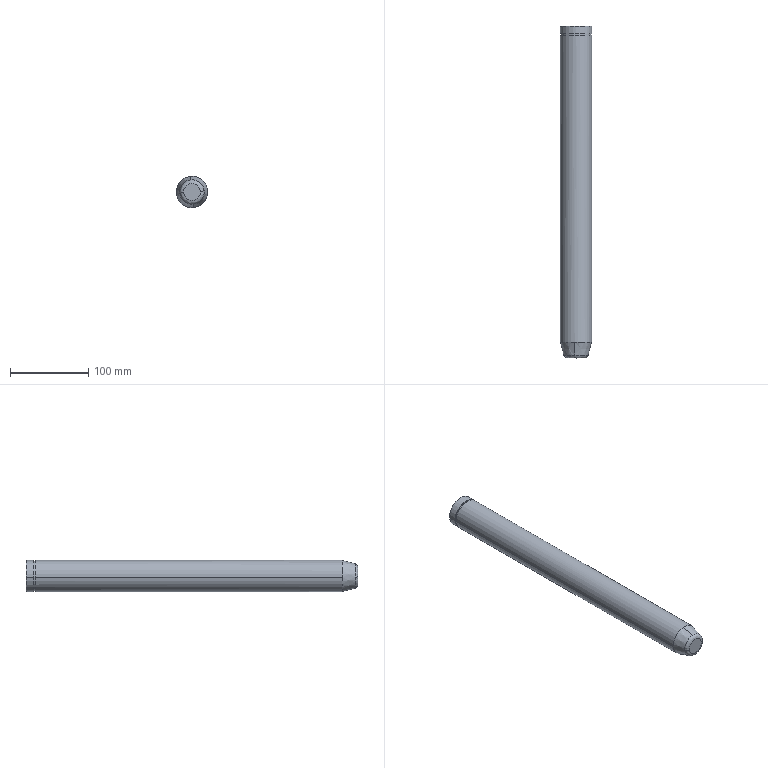Component | SolidWorks | YC1-250-05-02EjectorRod-1 | 1 solid | 14 faces | box 40 x 425 x 40 mm | volume 527461 mm3 | cylinder 6 | plane 4 | spline 2 | cone 2 | commonest cylinder face diameters 40 x4 38 x2 | material Plain Carbon Steel
STEP:
#1=CARTESIAN_POINT('',(-24.636,78.351,-0.05895));
#2=VERTEX_POINT('',#1);
#3=CARTESIAN_POINT('',(-23.789,78.351,0.01958));
#4=VERTEX_POINT('',#3);
#5=CARTESIAN_POINT('',(-24.636,78.351,-0.05895));
#6=CARTESIAN_POINT('',(-24.715,78.351,0.7882));
#7=CARTESIAN_POINT('',(-23.868,78.351,0.8667));
#8=CARTESIAN_POINT('',(-23.789,78.351,0.01958));
#9=(BOUNDED_CURVE()B_SPLINE_CURVE(3,(#5,#6,#7,#8),.UNSPECIFIED.,.F.,.F.)B_SPLINE_CURVE_WITH_KNOTS((4,4),(0.,1.),.UNSPECIFIED.)CURVE()GEOMETRIC_REPRESENTATION_ITEM()RATIONAL_B_SPLINE_CURVE((1.,0.3333,0.3333,1.))REPRESENTATION_ITEM(''));
#10=EDGE_CURVE('',#2,#4,#9,.T.);
#11=ORIENTED_EDGE('',*,*,#10,.T.);
#12=CARTESIAN_POINT('',(-23.6,78.497,0.03714));
#13=VERTEX_POINT('',#12);
#14=CARTESIAN_POINT('',(-23.789,78.547,0.01958));
#15=DIRECTION('',(-0.09232,0.,0.9957));
#16=DIRECTION('',(0.9957,0.,0.09232));
#17=AXIS2_PLACEMENT_3D('',#14,#15,#16);
#18=CIRCLE('',#17,0.1969);
#19=EDGE_CURVE('',#4,#13,#18,.T.);
#20=ORIENTED_EDGE('',*,*,#19,.T.);
#21=CARTESIAN_POINT('',(-24.269,78.497,0.5932));
#22=VERTEX_POINT('',#21);
#23=CARTESIAN_POINT('',(-24.213,78.497,-0.01969));
#24=DIRECTION('',(0.,1.,0.));
#25=DIRECTION('',(0.9957,0.,0.09232));
#26=AXIS2_PLACEMENT_3D('',#23,#24,#25);
#27=CIRCLE('',#26,0.6155);
#28=EDGE_CURVE('',#22,#13,#27,.T.);
#29=ORIENTED_EDGE('',*,*,#28,.F.);
#30=CARTESIAN_POINT('',(-24.825,78.497,-0.07651));
#31=VERTEX_POINT('',#30);
#32=CARTESIAN_POINT('',(-24.213,78.497,-0.01969));
#33=DIRECTION('',(0.,1.,0.));
#34=DIRECTION('',(0.9957,0.,0.09232));
#35=AXIS2_PLACEMENT_3D('',#32,#33,#34);
#36=CIRCLE('',#35,0.6155);
#37=EDGE_CURVE('',#31,#22,#36,.T.);
#38=ORIENTED_EDGE('',*,*,#37,.F.);
#39=CARTESIAN_POINT('',(-24.636,78.547,-0.05895));
#40=DIRECTION('',(0.09232,0.,-0.9957));
#41=DIRECTION('',(-0.9957,0.,-0.09232));
#42=AXIS2_PLACEMENT_3D('',#39,#40,#41);
#43=CIRCLE('',#42,0.1969);
#44=EDGE_CURVE('',#2,#31,#43,.T.);
#45=ORIENTED_EDGE('',*,*,#44,.F.);
#46=EDGE_LOOP('',(#11,#20,#29,#38,#45));
#47=FACE_OUTER_BOUND('',#46,.T.);
#48=CARTESIAN_POINT('',(-23.789,78.351,0.01958));
#49=CARTESIAN_POINT('',(-23.868,78.351,0.8667));
#50=CARTESIAN_POINT('',(-24.715,78.351,0.7882));
#51=CARTESIAN_POINT('',(-24.636,78.351,-0.05895));
#52=CARTESIAN_POINT('',(-23.697,78.351,0.02814));
#53=CARTESIAN_POINT('',(-23.792,78.351,1.06));
#54=CARTESIAN_POINT('',(-24.824,78.351,0.9641));
#55=CARTESIAN_POINT('',(-24.728,78.351,-0.06751));
#56=CARTESIAN_POINT('',(-23.624,78.407,0.03492));
#57=CARTESIAN_POINT('',(-23.733,78.407,1.213));
#58=CARTESIAN_POINT('',(-24.911,78.407,1.104));
#59=CARTESIAN_POINT('',(-24.802,78.407,-0.07429));
#60=CARTESIAN_POINT('',(-23.6,78.497,0.03714));
#61=CARTESIAN_POINT('',(-23.713,78.497,1.263));
#62=CARTESIAN_POINT('',(-24.939,78.497,1.149));
#63=CARTESIAN_POINT('',(-24.825,78.497,-0.07651));
#64=(BOUNDED_SURFACE()B_SPLINE_SURFACE(3,3,((#48,#49,#50,#51),(#52,#53,#54,#55),(#56,#57,#58,#59),(#60,#61,#62,#63)),.UNSPECIFIED.,.F.,.F.,.F.)B_SPLINE_SURFACE_WITH_KNOTS((4,4),(4,4),(0.,1.),(0.,1.),.UNSPECIFIED.)GEOMETRIC_REPRESENTATION_ITEM()RATIONAL_B_SPLINE_SURFACE(((1.,0.3333,0.3333,1.),(0.8622,0.2874,0.2874,0.8622),(0.8622,0.2874,0.2874,0.8622),(1.,0.3333,0.3333,1.)))REPRESENTATION_ITEM('')SURFACE());
#65=ADVANCED_FACE('',(#47),#64,.T.);
#66=CARTESIAN_POINT('',(-24.997,94.614,-0.09237));
#67=VERTEX_POINT('',#66);
#68=CARTESIAN_POINT('',(-23.429,94.614,0.053));
#69=VERTEX_POINT('',#68);
#70=CARTESIAN_POINT('',(-24.213,94.614,-0.01969));
#71=DIRECTION('',(0.,-1.,0.));
#72=DIRECTION('',(-0.9957,0.,-0.09232));
#73=AXIS2_PLACEMENT_3D('',#70,#71,#72);
#74=CIRCLE('',#73,0.7874);
#75=EDGE_CURVE('',#67,#69,#74,.T.);
#76=ORIENTED_EDGE('',*,*,#75,.T.);
#77=CARTESIAN_POINT('',(-23.429,79.138,0.053));
#78=VERTEX_POINT('',#77);
#79=CARTESIAN_POINT('',(-23.429,78.351,0.053));
#80=DIRECTION('',(0.,-1.,0.));
#81=VECTOR('',#80,39.37);
#82=LINE('',#79,#81);
#83=EDGE_CURVE('',#69,#78,#82,.T.);
#84=ORIENTED_EDGE('',*,*,#83,.T.);
#85=CARTESIAN_POINT('',(-24.14,79.138,-0.8037));
#86=VERTEX_POINT('',#85);
#87=CARTESIAN_POINT('',(-24.213,79.138,-0.01969));
#88=DIRECTION('',(0.,1.,0.));
#89=DIRECTION('',(-0.9957,0.,-0.09232));
#90=AXIS2_PLACEMENT_3D('',#87,#88,#89);
#91=CIRCLE('',#90,0.7874);
#92=EDGE_CURVE('',#78,#86,#91,.T.);
#93=ORIENTED_EDGE('',*,*,#92,.T.);
#94=CARTESIAN_POINT('',(-24.997,79.138,-0.09237));
#95=VERTEX_POINT('',#94);
#96=CARTESIAN_POINT('',(-24.213,79.138,-0.01969));
#97=DIRECTION('',(0.,1.,0.));
#98=DIRECTION('',(-0.9957,0.,-0.09232));
#99=AXIS2_PLACEMENT_3D('',#96,#97,#98);
#100=CIRCLE('',#99,0.7874);
#101=EDGE_CURVE('',#86,#95,#100,.T.);
#102=ORIENTED_EDGE('',*,*,#101,.T.);
#103=CARTESIAN_POINT('',(-24.997,78.351,-0.09237));
#104=DIRECTION('',(0.,-1.,0.));
#105=VECTOR('',#104,39.37);
#106=LINE('',#103,#105);
#107=EDGE_CURVE('',#67,#95,#106,.T.);
#108=ORIENTED_EDGE('',*,*,#107,.F.);
#109=EDGE_LOOP('',(#76,#84,#93,#102,#108));
#110=FACE_OUTER_BOUND('',#109,.T.);
#111=CARTESIAN_POINT('',(-24.213,78.351,-0.01969));
#112=DIRECTION('',(0.,-1.,0.));
#113=DIRECTION('',(-0.9957,0.,-0.09232));
#114=AXIS2_PLACEMENT_3D('',#111,#112,#113);
#115=CYLINDRICAL_SURFACE('',#114,0.7874);
#116=ADVANCED_FACE('',(#110),#115,.T.);
#117=ORIENTED_EDGE('',*,*,#28,.T.);
#118=CARTESIAN_POINT('',(-24.156,78.497,-0.6326));
#119=VERTEX_POINT('',#118);
#120=CARTESIAN_POINT('',(-24.213,78.497,-0.01969));
#121=DIRECTION('',(0.,1.,0.));
#122=DIRECTION('',(0.9957,0.,0.09232));
#123=AXIS2_PLACEMENT_3D('',#120,#121,#122);
#124=CIRCLE('',#123,0.6155);
#125=EDGE_CURVE('',#13,#119,#124,.T.);
#126=ORIENTED_EDGE('',*,*,#125,.T.);
#127=CARTESIAN_POINT('',(-24.14,79.138,-0.8037));
#128=DIRECTION('',(0.02389,0.9659,-0.2577));
#129=VECTOR('',#128,39.37);
#130=LINE('',#127,#129);
#131=EDGE_CURVE('',#119,#86,#130,.T.);
#132=ORIENTED_EDGE('',*,*,#131,.T.);
#133=ORIENTED_EDGE('',*,*,#92,.F.);
#134=CARTESIAN_POINT('',(-24.285,79.138,0.7644));
#135=VERTEX_POINT('',#134);
#136=CARTESIAN_POINT('',(-24.213,79.138,-0.01969));
#137=DIRECTION('',(0.,1.,0.));
#138=DIRECTION('',(-0.9957,0.,-0.09232));
#139=AXIS2_PLACEMENT_3D('',#136,#137,#138);
#140=CIRCLE('',#139,0.7874);
#141=EDGE_CURVE('',#135,#78,#140,.T.);
#142=ORIENTED_EDGE('',*,*,#141,.F.);
#143=CARTESIAN_POINT('',(-24.285,79.138,0.7644));
#144=DIRECTION('',(-0.02389,0.9659,0.2577));
#145=VECTOR('',#144,39.37);
#146=LINE('',#143,#145);
#147=EDGE_CURVE('',#22,#135,#146,.T.);
#148=ORIENTED_EDGE('',*,*,#147,.F.);
#149=EDGE_LOOP('',(#117,#126,#132,#133,#142,#148));
#150=FACE_OUTER_BOUND('',#149,.T.);
#151=CARTESIAN_POINT('',(-24.213,79.138,-0.01969));
#152=DIRECTION('',(0.,1.,-0.));
#153=DIRECTION('',(-0.09232,0.,0.9957));
#154=AXIS2_PLACEMENT_3D('',#151,#152,#153);
#155=CONICAL_SURFACE('',#154,0.7874,0.2618);
#156=ADVANCED_FACE('',(#150),#155,.T.);
#157=CARTESIAN_POINT('',(-24.957,94.689,-0.08874));
#158=VERTEX_POINT('',#157);
#159=CARTESIAN_POINT('',(-23.468,94.689,0.04937));
#160=VERTEX_POINT('',#159);
#161=CARTESIAN_POINT('',(-24.213,94.689,-0.01969));
#162=DIRECTION('',(0.,-1.,0.));
#163=DIRECTION('',(-0.9957,0.,-0.09232));
#164=AXIS2_PLACEMENT_3D('',#161,#162,#163);
#165=CIRCLE('',#164,0.748);
#166=EDGE_CURVE('',#158,#160,#165,.T.);
#167=ORIENTED_EDGE('',*,*,#166,.T.);
#168=CARTESIAN_POINT('',(-23.468,94.614,0.04937));
#169=VERTEX_POINT('',#168);
#170=CARTESIAN_POINT('',(-23.468,78.351,0.04937));
#171=DIRECTION('',(0.,-1.,0.));
#172=VECTOR('',#171,39.37);
#173=LINE('',#170,#172);
#174=EDGE_CURVE('',#160,#169,#173,.T.);
#175=ORIENTED_EDGE('',*,*,#174,.T.);
#176=CARTESIAN_POINT('',(-24.957,94.614,-0.08874));
#177=VERTEX_POINT('',#176);
#178=CARTESIAN_POINT('',(-24.213,94.614,-0.01969));
#179=DIRECTION('',(0.,1.,0.));
#180=DIRECTION('',(-0.9957,0.,-0.09232));
#181=AXIS2_PLACEMENT_3D('',#178,#179,#180);
#182=CIRCLE('',#181,0.748);
#183=EDGE_CURVE('',#169,#177,#182,.T.);
#184=ORIENTED_EDGE('',*,*,#183,.T.);
#185=CARTESIAN_POINT('',(-24.957,78.351,-0.08874));
#186=DIRECTION('',(0.,-1.,0.));
#187=VECTOR('',#186,39.37);
#188=LINE('',#185,#187);
#189=EDGE_CURVE('',#158,#177,#188,.T.);
#190=ORIENTED_EDGE('',*,*,#189,.F.);
#191=EDGE_LOOP('',(#167,#175,#184,#190));
#192=FACE_OUTER_BOUND('',#191,.T.);
#193=CARTESIAN_POINT('',(-24.213,78.351,-0.01969));
#194=DIRECTION('',(0.,-1.,0.));
#195=DIRECTION('',(-0.9957,0.,-0.09232));
#196=AXIS2_PLACEMENT_3D('',#193,#194,#195);
#197=CYLINDRICAL_SURFACE('',#196,0.748);
#198=ADVANCED_FACE('',(#192),#197,.T.);
#199=CARTESIAN_POINT('',(-24.997,95.083,-0.09237));
#200=VERTEX_POINT('',#199);
#201=CARTESIAN_POINT('',(-23.429,95.083,0.053));
#202=VERTEX_POINT('',#201);
#203=CARTESIAN_POINT('',(-24.213,95.083,-0.01969));
#204=DIRECTION('',(0.,-1.,0.));
#205=DIRECTION('',(-0.9957,0.,-0.09232));
#206=AXIS2_PLACEMENT_3D('',#203,#204,#205);
#207=CIRCLE('',#206,0.7874);
#208=EDGE_CURVE('',#200,#202,#207,.T.);
#209=ORIENTED_EDGE('',*,*,#208,.T.);
#210=CARTESIAN_POINT('',(-23.429,94.689,0.053));
#211=VERTEX_POINT('',#210);
#212=CARTESIAN_POINT('',(-23.429,78.351,0.053));
#213=DIRECTION('',(0.,-1.,0.));
#214=VECTOR('',#213,39.37);
#215=LINE('',#212,#214);
#216=EDGE_CURVE('',#202,#211,#215,.T.);
#217=ORIENTED_EDGE('',*,*,#216,.T.);
#218=CARTESIAN_POINT('',(-24.997,94.689,-0.09237));
#219=VERTEX_POINT('',#218);
#220=CARTESIAN_POINT('',(-24.213,94.689,-0.01969));
#221=DIRECTION('',(0.,1.,0.));
#222=DIRECTION('',(-0.9957,0.,-0.09232));
#223=AXIS2_PLACEMENT_3D('',#220,#221,#222);
#224=CIRCLE('',#223,0.7874);
#225=EDGE_CURVE('',#211,#219,#224,.T.);
#226=ORIENTED_EDGE('',*,*,#225,.T.);
#227=CARTESIAN_POINT('',(-24.997,78.351,-0.09237));
#228=DIRECTION('',(0.,-1.,0.));
#229=VECTOR('',#228,39.37);
#230=LINE('',#227,#229);
#231=EDGE_CURVE('',#200,#219,#230,.T.);
#232=ORIENTED_EDGE('',*,*,#231,.F.);
#233=EDGE_LOOP('',(#209,#217,#226,#232));
#234=FACE_OUTER_BOUND('',#233,.T.);
#235=CARTESIAN_POINT('',(-24.213,78.351,-0.01969));
#236=DIRECTION('',(0.,-1.,0.));
#237=DIRECTION('',(-0.9957,0.,-0.09232));
#238=AXIS2_PLACEMENT_3D('',#235,#236,#237);
#239=CYLINDRICAL_SURFACE('',#238,0.7874);
#240=ADVANCED_FACE('',(#234),#239,.T.);
#241=ORIENTED_EDGE('',*,*,#83,.F.);
#242=CARTESIAN_POINT('',(-24.213,94.614,-0.01969));
#243=DIRECTION('',(0.,-1.,0.));
#244=DIRECTION('',(-0.9957,0.,-0.09232));
#245=AXIS2_PLACEMENT_3D('',#242,#243,#244);
#246=CIRCLE('',#245,0.7874);
#247=EDGE_CURVE('',#69,#67,#246,.T.);
#248=ORIENTED_EDGE('',*,*,#247,.T.);
#249=ORIENTED_EDGE('',*,*,#107,.T.);
#250=CARTESIAN_POINT('',(-24.213,79.138,-0.01969));
#251=DIRECTION('',(0.,1.,0.));
#252=DIRECTION('',(-0.9957,0.,-0.09232));
#253=AXIS2_PLACEMENT_3D('',#250,#251,#252);
#254=CIRCLE('',#253,0.7874);
#255=EDGE_CURVE('',#95,#135,#254,.T.);
#256=ORIENTED_EDGE('',*,*,#255,.T.);
#257=ORIENTED_EDGE('',*,*,#141,.T.);
#258=EDGE_LOOP('',(#241,#248,#249,#256,#257));
#259=FACE_OUTER_BOUND('',#258,.T.);
#260=CARTESIAN_POINT('',(-24.213,78.351,-0.01969));
#261=DIRECTION('',(0.,-1.,0.));
#262=DIRECTION('',(-0.9957,0.,-0.09232));
#263=AXIS2_PLACEMENT_3D('',#260,#261,#262);
#264=CYLINDRICAL_SURFACE('',#263,0.7874);
#265=ADVANCED_FACE('',(#259),#264,.T.);
#266=ORIENTED_EDGE('',*,*,#131,.F.);
#267=CARTESIAN_POINT('',(-24.213,78.497,-0.01969));
#268=DIRECTION('',(0.,1.,0.));
#269=DIRECTION('',(0.9957,0.,0.09232));
#270=AXIS2_PLACEMENT_3D('',#267,#268,#269);
#271=CIRCLE('',#270,0.6155);
#272=EDGE_CURVE('',#119,#31,#271,.T.);
#273=ORIENTED_EDGE('',*,*,#272,.T.);
#274=ORIENTED_EDGE('',*,*,#37,.T.);
#275=ORIENTED_EDGE('',*,*,#147,.T.);
#276=ORIENTED_EDGE('',*,*,#255,.F.);
#277=ORIENTED_EDGE('',*,*,#101,.F.);
#278=EDGE_LOOP('',(#266,#273,#274,#275,#276,#277));
#279=FACE_OUTER_BOUND('',#278,.T.);
#280=CARTESIAN_POINT('',(-24.213,79.138,-0.01969));
#281=DIRECTION('',(0.,1.,-0.));
#282=DIRECTION('',(-0.09232,0.,0.9957));
#283=AXIS2_PLACEMENT_3D('',#280,#281,#282);
#284=CONICAL_SURFACE('',#283,0.7874,0.2618);
#285=ADVANCED_FACE('',(#279),#284,.T.);
#286=CARTESIAN_POINT('',(-24.213,94.614,-0.01969));
#287=DIRECTION('',(0.,1.,0.));
#288=DIRECTION('',(-0.9957,0.,-0.09232));
#289=AXIS2_PLACEMENT_3D('',#286,#287,#288);
#290=CIRCLE('',#289,0.748);
#291=EDGE_CURVE('',#177,#169,#290,.T.);
#292=ORIENTED_EDGE('',*,*,#291,.F.);
#293=ORIENTED_EDGE('',*,*,#183,.F.);
#294=EDGE_LOOP('',(#292,#293));
#295=FACE_BOUND('',#294,.T.);
#296=ORIENTED_EDGE('',*,*,#75,.F.);
#297=ORIENTED_EDGE('',*,*,#247,.F.);
#298=EDGE_LOOP('',(#296,#297));
#299=FACE_OUTER_BOUND('',#298,.T.);
#300=CARTESIAN_POINT('',(-24.144,94.614,-0.7645));
#301=DIRECTION('',(0.,-1.,0.));
#302=DIRECTION('',(-0.9957,0.,-0.09232));
#303=AXIS2_PLACEMENT_3D('',#300,#301,#302);
#304=PLANE('',#303);
#305=ADVANCED_FACE('',(#295,#299),#304,.F.);
#306=ORIENTED_EDGE('',*,*,#19,.F.);
#307=CARTESIAN_POINT('',(-23.789,78.351,0.01958));
#308=CARTESIAN_POINT('',(-23.711,78.351,-0.8275));
#309=CARTESIAN_POINT('',(-24.558,78.351,-0.9061));
#310=CARTESIAN_POINT('',(-24.636,78.351,-0.05895));
#311=(BOUNDED_CURVE()B_SPLINE_CURVE(3,(#307,#308,#309,#310),.UNSPECIFIED.,.F.,.T.)B_SPLINE_CURVE_WITH_KNOTS((4,4),(0.,1.),.UNSPECIFIED.)CURVE()GEOMETRIC_REPRESENTATION_ITEM()RATIONAL_B_SPLINE_CURVE((1.,0.3333,0.3333,1.))REPRESENTATION_ITEM(''));
#312=EDGE_CURVE('',#4,#2,#311,.T.);
#313=ORIENTED_EDGE('',*,*,#312,.T.);
#314=ORIENTED_EDGE('',*,*,#44,.T.);
#315=ORIENTED_EDGE('',*,*,#272,.F.);
#316=ORIENTED_EDGE('',*,*,#125,.F.);
#317=EDGE_LOOP('',(#306,#313,#314,#315,#316));
#318=FACE_OUTER_BOUND('',#317,.T.);
#319=CARTESIAN_POINT('',(-24.636,78.351,-0.05895));
#320=CARTESIAN_POINT('',(-24.558,78.351,-0.9061));
#321=CARTESIAN_POINT('',(-23.711,78.351,-0.8275));
#322=CARTESIAN_POINT('',(-23.789,78.351,0.01958));
#323=CARTESIAN_POINT('',(-24.728,78.351,-0.06751));
#324=CARTESIAN_POINT('',(-24.633,78.351,-1.099));
#325=CARTESIAN_POINT('',(-23.601,78.351,-1.003));
#326=CARTESIAN_POINT('',(-23.697,78.351,0.02814));
#327=CARTESIAN_POINT('',(-24.802,78.407,-0.07429));
#328=CARTESIAN_POINT('',(-24.692,78.407,-1.252));
#329=CARTESIAN_POINT('',(-23.514,78.407,-1.143));
#330=CARTESIAN_POINT('',(-23.624,78.407,0.03492));
#331=CARTESIAN_POINT('',(-24.825,78.497,-0.07651));
#332=CARTESIAN_POINT('',(-24.712,78.497,-1.302));
#333=CARTESIAN_POINT('',(-23.486,78.497,-1.189));
#334=CARTESIAN_POINT('',(-23.6,78.497,0.03714));
#335=(BOUNDED_SURFACE()B_SPLINE_SURFACE(3,3,((#319,#320,#321,#322),(#323,#324,#325,#326),(#327,#328,#329,#330),(#331,#332,#333,#334)),.UNSPECIFIED.,.F.,.F.,.F.)B_SPLINE_SURFACE_WITH_KNOTS((4,4),(4,4),(0.,1.),(0.,1.),.UNSPECIFIED.)GEOMETRIC_REPRESENTATION_ITEM()RATIONAL_B_SPLINE_SURFACE(((1.,0.3333,0.3333,1.),(0.8622,0.2874,0.2874,0.8622),(0.8622,0.2874,0.2874,0.8622),(1.,0.3333,0.3333,1.)))REPRESENTATION_ITEM('')SURFACE());
#336=ADVANCED_FACE('',(#318),#335,.T.);
#337=ORIENTED_EDGE('',*,*,#174,.F.);
#338=CARTESIAN_POINT('',(-24.213,94.689,-0.01969));
#339=DIRECTION('',(0.,-1.,0.));
#340=DIRECTION('',(-0.9957,0.,-0.09232));
#341=AXIS2_PLACEMENT_3D('',#338,#339,#340);
#342=CIRCLE('',#341,0.748);
#343=EDGE_CURVE('',#160,#158,#342,.T.);
#344=ORIENTED_EDGE('',*,*,#343,.T.);
#345=ORIENTED_EDGE('',*,*,#189,.T.);
#346=ORIENTED_EDGE('',*,*,#291,.T.);
#347=EDGE_LOOP('',(#337,#344,#345,#346));
#348=FACE_OUTER_BOUND('',#347,.T.);
#349=CARTESIAN_POINT('',(-24.213,78.351,-0.01969));
#350=DIRECTION('',(0.,-1.,0.));
#351=DIRECTION('',(-0.9957,0.,-0.09232));
#352=AXIS2_PLACEMENT_3D('',#349,#350,#351);
#353=CYLINDRICAL_SURFACE('',#352,0.748);
#354=ADVANCED_FACE('',(#348),#353,.T.);
#355=ORIENTED_EDGE('',*,*,#312,.F.);
#356=ORIENTED_EDGE('',*,*,#10,.F.);
#357=EDGE_LOOP('',(#355,#356));
#358=FACE_OUTER_BOUND('',#357,.T.);
#359=CARTESIAN_POINT('',(-24.213,78.351,-0.01969));
#360=DIRECTION('',(0.,-1.,0.));
#361=DIRECTION('',(-0.9957,0.,-0.09232));
#362=AXIS2_PLACEMENT_3D('',#359,#360,#361);
#363=PLANE('',#362);
#364=ADVANCED_FACE('',(#358),#363,.T.);
#365=CARTESIAN_POINT('',(-24.213,94.689,-0.01969));
#366=DIRECTION('',(0.,1.,0.));
#367=DIRECTION('',(-0.9957,0.,-0.09232));
#368=AXIS2_PLACEMENT_3D('',#365,#366,#367);
#369=CIRCLE('',#368,0.7874);
#370=EDGE_CURVE('',#219,#211,#369,.T.);
#371=ORIENTED_EDGE('',*,*,#370,.F.);
#372=ORIENTED_EDGE('',*,*,#225,.F.);
#373=EDGE_LOOP('',(#371,#372));
#374=FACE_OUTER_BOUND('',#373,.T.);
#375=ORIENTED_EDGE('',*,*,#166,.F.);
#376=ORIENTED_EDGE('',*,*,#343,.F.);
#377=EDGE_LOOP('',(#375,#376));
#378=FACE_BOUND('',#377,.T.);
#379=CARTESIAN_POINT('',(-24.144,94.689,-0.7645));
#380=DIRECTION('',(0.,1.,0.));
#381=DIRECTION('',(0.9957,0.,0.09232));
#382=AXIS2_PLACEMENT_3D('',#379,#380,#381);
#383=PLANE('',#382);
#384=ADVANCED_FACE('',(#374,#378),#383,.F.);
#385=ORIENTED_EDGE('',*,*,#216,.F.);
#386=CARTESIAN_POINT('',(-24.213,95.083,-0.01969));
#387=DIRECTION('',(0.,-1.,0.));
#388=DIRECTION('',(-0.9957,0.,-0.09232));
#389=AXIS2_PLACEMENT_3D('',#386,#387,#388);
#390=CIRCLE('',#389,0.7874);
#391=EDGE_CURVE('',#202,#200,#390,.T.);
#392=ORIENTED_EDGE('',*,*,#391,.T.);
#393=ORIENTED_EDGE('',*,*,#231,.T.);
#394=ORIENTED_EDGE('',*,*,#370,.T.);
#395=EDGE_LOOP('',(#385,#392,#393,#394));
#396=FACE_OUTER_BOUND('',#395,.T.);
#397=CARTESIAN_POINT('',(-24.213,78.351,-0.01969));
#398=DIRECTION('',(0.,-1.,0.));
#399=DIRECTION('',(-0.9957,0.,-0.09232));
#400=AXIS2_PLACEMENT_3D('',#397,#398,#399);
#401=CYLINDRICAL_SURFACE('',#400,0.7874);
#402=ADVANCED_FACE('',(#396),#401,.T.);
#403=ORIENTED_EDGE('',*,*,#208,.F.);
#404=ORIENTED_EDGE('',*,*,#391,.F.);
#405=EDGE_LOOP('',(#403,#404));
#406=FACE_OUTER_BOUND('',#405,.T.);
#407=CARTESIAN_POINT('',(-24.14,95.083,-0.8037));
#408=DIRECTION('',(0.,1.,0.));
#409=DIRECTION('',(0.9957,0.,0.09232));
#410=AXIS2_PLACEMENT_3D('',#407,#408,#409);
#411=PLANE('',#410);
#412=ADVANCED_FACE('',(#406),#411,.T.);
#413=CLOSED_SHELL('',(#65,#116,#156,#198,#240,#265,#285,#305,#336,#354,#364,#384,#402,#412));
#414=MANIFOLD_SOLID_BREP('',#413);
#415=CARTESIAN_POINT('',(0.,0.,0.));
#416=DIRECTION('',(0.,0.,1.));
#417=DIRECTION('',(1.,0.,0.));
#418=AXIS2_PLACEMENT_3D('',#415,#416,#417);
#419=(LENGTH_UNIT()NAMED_UNIT(*)SI_UNIT($,.METRE.));
#420=LENGTH_MEASURE_WITH_UNIT(LENGTH_MEASURE(0.0254),#419);
#421=DIMENSIONAL_EXPONENTS(1.,0.,0.,0.,0.,0.,0.);
#422=(CONVERSION_BASED_UNIT('',#420)LENGTH_UNIT()NAMED_UNIT(#421));
#423=UNCERTAINTY_MEASURE_WITH_UNIT(LENGTH_MEASURE(0.00001),#422,'','');
#424=(NAMED_UNIT(*)PLANE_ANGLE_UNIT()SI_UNIT($,.RADIAN.));
#425=(NAMED_UNIT(*)SI_UNIT($,.STERADIAN.)SOLID_ANGLE_UNIT());
#426=(GEOMETRIC_REPRESENTATION_CONTEXT(3)GLOBAL_UNCERTAINTY_ASSIGNED_CONTEXT((#423))GLOBAL_UNIT_ASSIGNED_CONTEXT((#422,#424,#425))REPRESENTATION_CONTEXT('',''));
#427=ADVANCED_BREP_SHAPE_REPRESENTATION('',(#414,#418),#426);
#428=COLOUR_RGB('',0.7922,0.8196,0.9333);
#429=FILL_AREA_STYLE_COLOUR('',#428);
#430=FILL_AREA_STYLE('',(#429));
#431=SURFACE_STYLE_FILL_AREA(#430);
#432=SURFACE_SIDE_STYLE('',(#431));
#433=SURFACE_STYLE_USAGE(.BOTH.,#432);
#434=PRESENTATION_STYLE_ASSIGNMENT((#433));
#435=STYLED_ITEM('',(#434),#414);
#436=PRESENTATION_LAYER_ASSIGNMENT('','',(#435));
#437=(LENGTH_UNIT()NAMED_UNIT(*)SI_UNIT($,.METRE.));
#438=LENGTH_MEASURE_WITH_UNIT(LENGTH_MEASURE(0.0254),#437);
#439=DIMENSIONAL_EXPONENTS(1.,0.,0.,0.,0.,0.,0.);
#440=(CONVERSION_BASED_UNIT('',#438)LENGTH_UNIT()NAMED_UNIT(#439));
#441=UNCERTAINTY_MEASURE_WITH_UNIT(LENGTH_MEASURE(0.00001),#440,'','');
#442=(NAMED_UNIT(*)PLANE_ANGLE_UNIT()SI_UNIT($,.RADIAN.));
#443=(NAMED_UNIT(*)SI_UNIT($,.STERADIAN.)SOLID_ANGLE_UNIT());
#444=(GEOMETRIC_REPRESENTATION_CONTEXT(3)GLOBAL_UNCERTAINTY_ASSIGNED_CONTEXT((#441))GLOBAL_UNIT_ASSIGNED_CONTEXT((#440,#442,#443))REPRESENTATION_CONTEXT('',''));
#445=MECHANICAL_DESIGN_GEOMETRIC_PRESENTATION_REPRESENTATION('',(#435),#444);